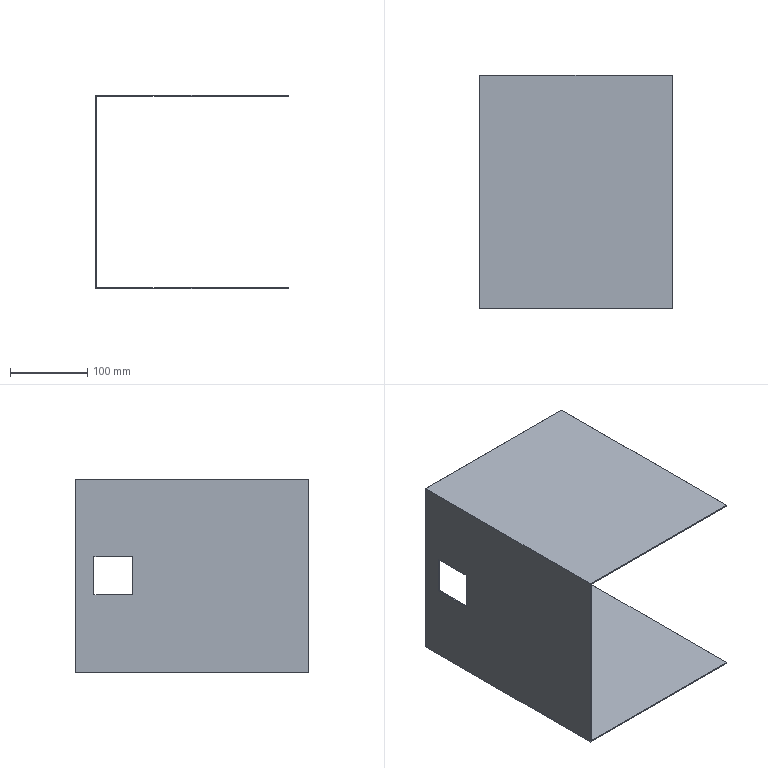Component | SolidWorks | InfraredProcessingChamber-1 | 1 solid | 14 faces | box 248.5 x 301 x 250 mm | volume 332222 mm3 | plane 14
build123d program:
from build123d import *

# Parameters (mm, degrees)
SKETCH1_W           = 250
SKETCH1_H           = 250
BOSS_EXTRUDE1_DEPTH = 301
SHELL1_T            = -1.5
SKETCH6_W           = 250
SKETCH6_H           = 301
CUT_EXTRUDE3_DEPTH  = 1.5
SKETCH7_W           = 49.25
SKETCH7_H           = 50
CUT_EXTRUDE4_DEPTH  = 1.5
SKETCH2_W           = 247
SKETCH2_H           = 247
CUT_EXTRUDE1_DEPTH  = 10


with BuildPart() as part:
    # Sketch1 → Boss-Extrude1 (new body)
    with BuildSketch(Plane(origin=(0, 0, 0), x_dir=(1, 0, 0), z_dir=(0, 1, 0))):
        Rectangle(SKETCH1_W, SKETCH1_H)
    extrude(amount=BOSS_EXTRUDE1_DEPTH)

    # Shell1
    shell1_openings = [part.faces().sort_by_distance(p)[0] for p in [
        (0, 0, 0),
    ]]
    offset(amount=SHELL1_T, openings=shell1_openings, kind=Kind.INTERSECTION)

    # Sketch6 → Cut-Extrude3 (cut)
    with BuildSketch(Plane.XY.offset(-123.5)):
        with Locations((0, 150.5)):
            Rectangle(SKETCH6_W, SKETCH6_H)
    extrude(amount=-CUT_EXTRUDE3_DEPTH, mode=Mode.SUBTRACT)

    # Sketch7 → Cut-Extrude4 (cut)
    with BuildSketch(Plane.XY.offset(125)):
        with Locations((0.375, 252)):
            Rectangle(SKETCH7_W, SKETCH7_H)
    extrude(amount=-CUT_EXTRUDE4_DEPTH, mode=Mode.SUBTRACT)

    # Sketch2 → Cut-Extrude1 (cut)
    with BuildSketch(Plane.XZ.offset(-299.5)):
        Rectangle(SKETCH2_W, SKETCH2_H)
    extrude(amount=-CUT_EXTRUDE1_DEPTH, mode=Mode.SUBTRACT)


solid = part.part

# Placed as in the assembly
solid = solid.moved(Location((175, 270, 0), (0, -90, 0)))
STEP:
#1=CARTESIAN_POINT('',(11.752,22.48,-4.862));
#2=VERTEX_POINT('',#1);
#3=CARTESIAN_POINT('',(11.752,22.48,-4.921));
#4=VERTEX_POINT('',#3);
#5=CARTESIAN_POINT('',(11.752,22.48,-4.921));
#6=DIRECTION('',(0.,0.,-1.));
#7=VECTOR('',#6,39.37);
#8=LINE('',#5,#7);
#9=EDGE_CURVE('',#2,#4,#8,.T.);
#10=ORIENTED_EDGE('',*,*,#9,.F.);
#11=CARTESIAN_POINT('',(11.752,10.63,-4.862));
#12=VERTEX_POINT('',#11);
#13=CARTESIAN_POINT('',(11.752,22.48,-4.862));
#14=DIRECTION('',(0.,-1.,0.));
#15=VECTOR('',#14,39.37);
#16=LINE('',#13,#15);
#17=EDGE_CURVE('',#2,#12,#16,.T.);
#18=ORIENTED_EDGE('',*,*,#17,.T.);
#19=CARTESIAN_POINT('',(11.752,10.63,-4.921));
#20=VERTEX_POINT('',#19);
#21=CARTESIAN_POINT('',(11.752,10.63,-4.921));
#22=DIRECTION('',(0.,0.,1.));
#23=VECTOR('',#22,39.37);
#24=LINE('',#21,#23);
#25=EDGE_CURVE('',#20,#12,#24,.T.);
#26=ORIENTED_EDGE('',*,*,#25,.F.);
#27=CARTESIAN_POINT('',(11.752,22.48,-4.921));
#28=DIRECTION('',(0.,-1.,0.));
#29=VECTOR('',#28,39.37);
#30=LINE('',#27,#29);
#31=EDGE_CURVE('',#4,#20,#30,.T.);
#32=ORIENTED_EDGE('',*,*,#31,.F.);
#33=EDGE_LOOP('',(#10,#18,#26,#32));
#34=FACE_OUTER_BOUND('',#33,.T.);
#35=CARTESIAN_POINT('',(11.752,10.63,0.));
#36=DIRECTION('',(-1.,0.,0.));
#37=DIRECTION('',(0.,0.,1.));
#38=AXIS2_PLACEMENT_3D('',#35,#36,#37);
#39=PLANE('',#38);
#40=ADVANCED_FACE('',(#34),#39,.F.);
#41=CARTESIAN_POINT('',(1.969,10.63,4.921));
#42=VERTEX_POINT('',#41);
#43=CARTESIAN_POINT('',(11.752,10.63,4.921));
#44=VERTEX_POINT('',#43);
#45=CARTESIAN_POINT('',(11.811,10.63,4.921));
#46=DIRECTION('',(1.,0.,0.));
#47=VECTOR('',#46,39.37);
#48=LINE('',#45,#47);
#49=EDGE_CURVE('',#42,#44,#48,.T.);
#50=ORIENTED_EDGE('',*,*,#49,.T.);
#51=CARTESIAN_POINT('',(11.752,22.48,4.921));
#52=VERTEX_POINT('',#51);
#53=CARTESIAN_POINT('',(11.752,22.48,4.921));
#54=DIRECTION('',(0.,1.,-0.));
#55=VECTOR('',#54,39.37);
#56=LINE('',#53,#55);
#57=EDGE_CURVE('',#44,#52,#56,.T.);
#58=ORIENTED_EDGE('',*,*,#57,.T.);
#59=CARTESIAN_POINT('',(1.969,22.48,4.921));
#60=VERTEX_POINT('',#59);
#61=CARTESIAN_POINT('',(11.811,22.48,4.921));
#62=DIRECTION('',(1.,0.,0.));
#63=VECTOR('',#62,39.37);
#64=LINE('',#61,#63);
#65=EDGE_CURVE('',#60,#52,#64,.T.);
#66=ORIENTED_EDGE('',*,*,#65,.F.);
#67=CARTESIAN_POINT('',(1.969,22.48,4.921));
#68=DIRECTION('',(0.,-1.,0.));
#69=VECTOR('',#68,39.37);
#70=LINE('',#67,#69);
#71=EDGE_CURVE('',#60,#42,#70,.T.);
#72=ORIENTED_EDGE('',*,*,#71,.T.);
#73=EDGE_LOOP('',(#50,#58,#66,#72));
#74=FACE_OUTER_BOUND('',#73,.T.);
#75=CARTESIAN_POINT('',(11.811,22.48,4.921));
#76=DIRECTION('',(0.,0.,-1.));
#77=DIRECTION('',(-1.,0.,0.));
#78=AXIS2_PLACEMENT_3D('',#75,#76,#77);
#79=PLANE('',#78);
#80=ADVANCED_FACE('',(#74),#79,.F.);
#81=CARTESIAN_POINT('',(1.969,22.48,-4.921));
#82=VERTEX_POINT('',#81);
#83=CARTESIAN_POINT('',(11.811,22.48,-4.921));
#84=DIRECTION('',(-1.,0.,0.));
#85=VECTOR('',#84,39.37);
#86=LINE('',#83,#85);
#87=EDGE_CURVE('',#4,#82,#86,.T.);
#88=ORIENTED_EDGE('',*,*,#87,.F.);
#89=ORIENTED_EDGE('',*,*,#31,.T.);
#90=CARTESIAN_POINT('',(1.969,10.63,-4.921));
#91=VERTEX_POINT('',#90);
#92=CARTESIAN_POINT('',(11.811,10.63,-4.921));
#93=DIRECTION('',(-1.,0.,0.));
#94=VECTOR('',#93,39.37);
#95=LINE('',#92,#94);
#96=EDGE_CURVE('',#20,#91,#95,.T.);
#97=ORIENTED_EDGE('',*,*,#96,.T.);
#98=CARTESIAN_POINT('',(1.969,22.48,-4.921));
#99=DIRECTION('',(0.,-1.,0.));
#100=VECTOR('',#99,39.37);
#101=LINE('',#98,#100);
#102=EDGE_CURVE('',#82,#91,#101,.T.);
#103=ORIENTED_EDGE('',*,*,#102,.F.);
#104=EDGE_LOOP('',(#88,#89,#97,#103));
#105=FACE_OUTER_BOUND('',#104,.T.);
#106=CARTESIAN_POINT('',(11.811,22.48,-4.921));
#107=DIRECTION('',(0.,0.,1.));
#108=DIRECTION('',(1.,0.,0.));
#109=AXIS2_PLACEMENT_3D('',#106,#107,#108);
#110=PLANE('',#109);
#111=ADVANCED_FACE('',(#105),#110,.F.);
#112=CARTESIAN_POINT('',(1.969,19.567,0.9843));
#113=VERTEX_POINT('',#112);
#114=CARTESIAN_POINT('',(1.969,21.535,0.9843));
#115=VERTEX_POINT('',#114);
#116=CARTESIAN_POINT('',(1.969,19.567,0.9843));
#117=DIRECTION('',(0.,1.,0.));
#118=VECTOR('',#117,39.37);
#119=LINE('',#116,#118);
#120=EDGE_CURVE('',#113,#115,#119,.T.);
#121=ORIENTED_EDGE('',*,*,#120,.F.);
#122=CARTESIAN_POINT('',(1.969,19.567,-0.9547));
#123=VERTEX_POINT('',#122);
#124=CARTESIAN_POINT('',(1.969,19.567,-0.9547));
#125=DIRECTION('',(0.,0.,1.));
#126=VECTOR('',#125,39.37);
#127=LINE('',#124,#126);
#128=EDGE_CURVE('',#123,#113,#127,.T.);
#129=ORIENTED_EDGE('',*,*,#128,.F.);
#130=CARTESIAN_POINT('',(1.969,21.535,-0.9547));
#131=VERTEX_POINT('',#130);
#132=CARTESIAN_POINT('',(1.969,21.535,-0.9547));
#133=DIRECTION('',(0.,-1.,0.));
#134=VECTOR('',#133,39.37);
#135=LINE('',#132,#134);
#136=EDGE_CURVE('',#131,#123,#135,.T.);
#137=ORIENTED_EDGE('',*,*,#136,.F.);
#138=CARTESIAN_POINT('',(1.969,21.535,0.9843));
#139=DIRECTION('',(0.,0.,-1.));
#140=VECTOR('',#139,39.37);
#141=LINE('',#138,#140);
#142=EDGE_CURVE('',#115,#131,#141,.T.);
#143=ORIENTED_EDGE('',*,*,#142,.F.);
#144=EDGE_LOOP('',(#121,#129,#137,#143));
#145=FACE_BOUND('',#144,.T.);
#146=CARTESIAN_POINT('',(1.969,10.63,-4.921));
#147=DIRECTION('',(0.,0.,1.));
#148=VECTOR('',#147,39.37);
#149=LINE('',#146,#148);
#150=EDGE_CURVE('',#91,#42,#149,.T.);
#151=ORIENTED_EDGE('',*,*,#150,.T.);
#152=ORIENTED_EDGE('',*,*,#71,.F.);
#153=CARTESIAN_POINT('',(1.969,22.48,-4.921));
#154=DIRECTION('',(0.,0.,1.));
#155=VECTOR('',#154,39.37);
#156=LINE('',#153,#155);
#157=EDGE_CURVE('',#82,#60,#156,.T.);
#158=ORIENTED_EDGE('',*,*,#157,.F.);
#159=ORIENTED_EDGE('',*,*,#102,.T.);
#160=EDGE_LOOP('',(#151,#152,#158,#159));
#161=FACE_OUTER_BOUND('',#160,.T.);
#162=CARTESIAN_POINT('',(1.969,22.48,-4.921));
#163=DIRECTION('',(1.,0.,0.));
#164=DIRECTION('',(0.,0.,-1.));
#165=AXIS2_PLACEMENT_3D('',#162,#163,#164);
#166=PLANE('',#165);
#167=ADVANCED_FACE('',(#145,#161),#166,.F.);
#168=CARTESIAN_POINT('',(2.028,22.48,-4.862));
#169=VERTEX_POINT('',#168);
#170=CARTESIAN_POINT('',(6.89,22.48,-4.862));
#171=DIRECTION('',(-1.,0.,0.));
#172=VECTOR('',#171,39.37);
#173=LINE('',#170,#172);
#174=EDGE_CURVE('',#2,#169,#173,.T.);
#175=ORIENTED_EDGE('',*,*,#174,.F.);
#176=ORIENTED_EDGE('',*,*,#9,.T.);
#177=ORIENTED_EDGE('',*,*,#87,.T.);
#178=ORIENTED_EDGE('',*,*,#157,.T.);
#179=ORIENTED_EDGE('',*,*,#65,.T.);
#180=CARTESIAN_POINT('',(11.752,22.48,4.862));
#181=VERTEX_POINT('',#180);
#182=CARTESIAN_POINT('',(11.752,22.48,-4.921));
#183=DIRECTION('',(0.,0.,-1.));
#184=VECTOR('',#183,39.37);
#185=LINE('',#182,#184);
#186=EDGE_CURVE('',#52,#181,#185,.T.);
#187=ORIENTED_EDGE('',*,*,#186,.T.);
#188=CARTESIAN_POINT('',(2.028,22.48,4.862));
#189=VERTEX_POINT('',#188);
#190=CARTESIAN_POINT('',(6.89,22.48,4.862));
#191=DIRECTION('',(1.,0.,0.));
#192=VECTOR('',#191,39.37);
#193=LINE('',#190,#192);
#194=EDGE_CURVE('',#189,#181,#193,.T.);
#195=ORIENTED_EDGE('',*,*,#194,.F.);
#196=CARTESIAN_POINT('',(2.028,22.48,0.));
#197=DIRECTION('',(0.,0.,1.));
#198=VECTOR('',#197,39.37);
#199=LINE('',#196,#198);
#200=EDGE_CURVE('',#169,#189,#199,.T.);
#201=ORIENTED_EDGE('',*,*,#200,.F.);
#202=EDGE_LOOP('',(#175,#176,#177,#178,#179,#187,#195,#201));
#203=FACE_OUTER_BOUND('',#202,.T.);
#204=CARTESIAN_POINT('',(6.89,22.48,0.));
#205=DIRECTION('',(0.,1.,0.));
#206=DIRECTION('',(-1.,0.,0.));
#207=AXIS2_PLACEMENT_3D('',#204,#205,#206);
#208=PLANE('',#207);
#209=ADVANCED_FACE('',(#203),#208,.T.);
#210=ORIENTED_EDGE('',*,*,#96,.F.);
#211=ORIENTED_EDGE('',*,*,#25,.T.);
#212=CARTESIAN_POINT('',(2.028,10.63,-4.862));
#213=VERTEX_POINT('',#212);
#214=CARTESIAN_POINT('',(11.811,10.63,-4.862));
#215=DIRECTION('',(-1.,0.,0.));
#216=VECTOR('',#215,39.37);
#217=LINE('',#214,#216);
#218=EDGE_CURVE('',#12,#213,#217,.T.);
#219=ORIENTED_EDGE('',*,*,#218,.T.);
#220=CARTESIAN_POINT('',(2.028,10.63,4.862));
#221=VERTEX_POINT('',#220);
#222=CARTESIAN_POINT('',(2.028,10.63,-4.921));
#223=DIRECTION('',(0.,0.,1.));
#224=VECTOR('',#223,39.37);
#225=LINE('',#222,#224);
#226=EDGE_CURVE('',#213,#221,#225,.T.);
#227=ORIENTED_EDGE('',*,*,#226,.T.);
#228=CARTESIAN_POINT('',(11.752,10.63,4.862));
#229=VERTEX_POINT('',#228);
#230=CARTESIAN_POINT('',(11.811,10.63,4.862));
#231=DIRECTION('',(1.,0.,0.));
#232=VECTOR('',#231,39.37);
#233=LINE('',#230,#232);
#234=EDGE_CURVE('',#221,#229,#233,.T.);
#235=ORIENTED_EDGE('',*,*,#234,.T.);
#236=CARTESIAN_POINT('',(11.752,10.63,-4.921));
#237=DIRECTION('',(0.,0.,1.));
#238=VECTOR('',#237,39.37);
#239=LINE('',#236,#238);
#240=EDGE_CURVE('',#229,#44,#239,.T.);
#241=ORIENTED_EDGE('',*,*,#240,.T.);
#242=ORIENTED_EDGE('',*,*,#49,.F.);
#243=ORIENTED_EDGE('',*,*,#150,.F.);
#244=EDGE_LOOP('',(#210,#211,#219,#227,#235,#241,#242,#243));
#245=FACE_OUTER_BOUND('',#244,.T.);
#246=CARTESIAN_POINT('',(6.89,10.63,0.));
#247=DIRECTION('',(0.,1.,0.));
#248=DIRECTION('',(-1.,0.,0.));
#249=AXIS2_PLACEMENT_3D('',#246,#247,#248);
#250=PLANE('',#249);
#251=ADVANCED_FACE('',(#245),#250,.F.);
#252=ORIENTED_EDGE('',*,*,#234,.F.);
#253=CARTESIAN_POINT('',(2.028,22.48,4.862));
#254=DIRECTION('',(0.,-1.,0.));
#255=VECTOR('',#254,39.37);
#256=LINE('',#253,#255);
#257=EDGE_CURVE('',#189,#221,#256,.T.);
#258=ORIENTED_EDGE('',*,*,#257,.F.);
#259=ORIENTED_EDGE('',*,*,#194,.T.);
#260=CARTESIAN_POINT('',(11.752,22.48,4.862));
#261=DIRECTION('',(0.,-1.,0.));
#262=VECTOR('',#261,39.37);
#263=LINE('',#260,#262);
#264=EDGE_CURVE('',#181,#229,#263,.T.);
#265=ORIENTED_EDGE('',*,*,#264,.T.);
#266=EDGE_LOOP('',(#252,#258,#259,#265));
#267=FACE_OUTER_BOUND('',#266,.T.);
#268=CARTESIAN_POINT('',(11.811,22.48,4.862));
#269=DIRECTION('',(0.,0.,-1.));
#270=DIRECTION('',(-1.,0.,0.));
#271=AXIS2_PLACEMENT_3D('',#268,#269,#270);
#272=PLANE('',#271);
#273=ADVANCED_FACE('',(#267),#272,.T.);
#274=ORIENTED_EDGE('',*,*,#218,.F.);
#275=ORIENTED_EDGE('',*,*,#17,.F.);
#276=ORIENTED_EDGE('',*,*,#174,.T.);
#277=CARTESIAN_POINT('',(2.028,22.48,-4.862));
#278=DIRECTION('',(0.,-1.,0.));
#279=VECTOR('',#278,39.37);
#280=LINE('',#277,#279);
#281=EDGE_CURVE('',#169,#213,#280,.T.);
#282=ORIENTED_EDGE('',*,*,#281,.T.);
#283=EDGE_LOOP('',(#274,#275,#276,#282));
#284=FACE_OUTER_BOUND('',#283,.T.);
#285=CARTESIAN_POINT('',(11.811,22.48,-4.862));
#286=DIRECTION('',(0.,0.,1.));
#287=DIRECTION('',(1.,0.,0.));
#288=AXIS2_PLACEMENT_3D('',#285,#286,#287);
#289=PLANE('',#288);
#290=ADVANCED_FACE('',(#284),#289,.T.);
#291=CARTESIAN_POINT('',(2.028,19.567,-0.9547));
#292=VERTEX_POINT('',#291);
#293=CARTESIAN_POINT('',(2.028,19.567,0.9843));
#294=VERTEX_POINT('',#293);
#295=CARTESIAN_POINT('',(2.028,19.567,-0.9547));
#296=DIRECTION('',(0.,0.,1.));
#297=VECTOR('',#296,39.37);
#298=LINE('',#295,#297);
#299=EDGE_CURVE('',#292,#294,#298,.T.);
#300=ORIENTED_EDGE('',*,*,#299,.T.);
#301=CARTESIAN_POINT('',(2.028,21.535,0.9843));
#302=VERTEX_POINT('',#301);
#303=CARTESIAN_POINT('',(2.028,19.567,0.9843));
#304=DIRECTION('',(0.,1.,0.));
#305=VECTOR('',#304,39.37);
#306=LINE('',#303,#305);
#307=EDGE_CURVE('',#294,#302,#306,.T.);
#308=ORIENTED_EDGE('',*,*,#307,.T.);
#309=CARTESIAN_POINT('',(2.028,21.535,-0.9547));
#310=VERTEX_POINT('',#309);
#311=CARTESIAN_POINT('',(2.028,21.535,0.9843));
#312=DIRECTION('',(0.,0.,-1.));
#313=VECTOR('',#312,39.37);
#314=LINE('',#311,#313);
#315=EDGE_CURVE('',#302,#310,#314,.T.);
#316=ORIENTED_EDGE('',*,*,#315,.T.);
#317=CARTESIAN_POINT('',(2.028,21.535,-0.9547));
#318=DIRECTION('',(0.,-1.,0.));
#319=VECTOR('',#318,39.37);
#320=LINE('',#317,#319);
#321=EDGE_CURVE('',#310,#292,#320,.T.);
#322=ORIENTED_EDGE('',*,*,#321,.T.);
#323=EDGE_LOOP('',(#300,#308,#316,#322));
#324=FACE_BOUND('',#323,.T.);
#325=ORIENTED_EDGE('',*,*,#226,.F.);
#326=ORIENTED_EDGE('',*,*,#281,.F.);
#327=ORIENTED_EDGE('',*,*,#200,.T.);
#328=ORIENTED_EDGE('',*,*,#257,.T.);
#329=EDGE_LOOP('',(#325,#326,#327,#328));
#330=FACE_OUTER_BOUND('',#329,.T.);
#331=CARTESIAN_POINT('',(2.028,22.48,-4.921));
#332=DIRECTION('',(1.,0.,0.));
#333=DIRECTION('',(0.,0.,-1.));
#334=AXIS2_PLACEMENT_3D('',#331,#332,#333);
#335=PLANE('',#334);
#336=ADVANCED_FACE('',(#324,#330),#335,.T.);
#337=ORIENTED_EDGE('',*,*,#264,.F.);
#338=ORIENTED_EDGE('',*,*,#186,.F.);
#339=ORIENTED_EDGE('',*,*,#57,.F.);
#340=ORIENTED_EDGE('',*,*,#240,.F.);
#341=EDGE_LOOP('',(#337,#338,#339,#340));
#342=FACE_OUTER_BOUND('',#341,.T.);
#343=CARTESIAN_POINT('',(11.752,10.63,0.));
#344=DIRECTION('',(-1.,0.,0.));
#345=DIRECTION('',(0.,0.,1.));
#346=AXIS2_PLACEMENT_3D('',#343,#344,#345);
#347=PLANE('',#346);
#348=ADVANCED_FACE('',(#342),#347,.F.);
#349=ORIENTED_EDGE('',*,*,#128,.T.);
#350=CARTESIAN_POINT('',(2.028,19.567,0.9843));
#351=DIRECTION('',(-1.,0.,0.));
#352=VECTOR('',#351,39.37);
#353=LINE('',#350,#352);
#354=EDGE_CURVE('',#294,#113,#353,.T.);
#355=ORIENTED_EDGE('',*,*,#354,.F.);
#356=ORIENTED_EDGE('',*,*,#299,.F.);
#357=CARTESIAN_POINT('',(2.028,19.567,-0.9547));
#358=DIRECTION('',(-1.,0.,0.));
#359=VECTOR('',#358,39.37);
#360=LINE('',#357,#359);
#361=EDGE_CURVE('',#292,#123,#360,.T.);
#362=ORIENTED_EDGE('',*,*,#361,.T.);
#363=EDGE_LOOP('',(#349,#355,#356,#362));
#364=FACE_OUTER_BOUND('',#363,.T.);
#365=CARTESIAN_POINT('',(2.028,19.567,-0.9547));
#366=DIRECTION('',(0.,-1.,0.));
#367=DIRECTION('',(1.,0.,0.));
#368=AXIS2_PLACEMENT_3D('',#365,#366,#367);
#369=PLANE('',#368);
#370=ADVANCED_FACE('',(#364),#369,.F.);
#371=ORIENTED_EDGE('',*,*,#136,.T.);
#372=ORIENTED_EDGE('',*,*,#361,.F.);
#373=ORIENTED_EDGE('',*,*,#321,.F.);
#374=CARTESIAN_POINT('',(2.028,21.535,-0.9547));
#375=DIRECTION('',(-1.,0.,0.));
#376=VECTOR('',#375,39.37);
#377=LINE('',#374,#376);
#378=EDGE_CURVE('',#310,#131,#377,.T.);
#379=ORIENTED_EDGE('',*,*,#378,.T.);
#380=EDGE_LOOP('',(#371,#372,#373,#379));
#381=FACE_OUTER_BOUND('',#380,.T.);
#382=CARTESIAN_POINT('',(2.028,21.535,-0.9547));
#383=DIRECTION('',(0.,-0.,-1.));
#384=DIRECTION('',(0.,-1.,0.));
#385=AXIS2_PLACEMENT_3D('',#382,#383,#384);
#386=PLANE('',#385);
#387=ADVANCED_FACE('',(#381),#386,.F.);
#388=ORIENTED_EDGE('',*,*,#142,.T.);
#389=ORIENTED_EDGE('',*,*,#378,.F.);
#390=ORIENTED_EDGE('',*,*,#315,.F.);
#391=CARTESIAN_POINT('',(2.028,21.535,0.9843));
#392=DIRECTION('',(-1.,0.,0.));
#393=VECTOR('',#392,39.37);
#394=LINE('',#391,#393);
#395=EDGE_CURVE('',#302,#115,#394,.T.);
#396=ORIENTED_EDGE('',*,*,#395,.T.);
#397=EDGE_LOOP('',(#388,#389,#390,#396));
#398=FACE_OUTER_BOUND('',#397,.T.);
#399=CARTESIAN_POINT('',(2.028,21.535,0.9843));
#400=DIRECTION('',(0.,1.,0.));
#401=DIRECTION('',(-1.,0.,0.));
#402=AXIS2_PLACEMENT_3D('',#399,#400,#401);
#403=PLANE('',#402);
#404=ADVANCED_FACE('',(#398),#403,.F.);
#405=ORIENTED_EDGE('',*,*,#120,.T.);
#406=ORIENTED_EDGE('',*,*,#395,.F.);
#407=ORIENTED_EDGE('',*,*,#307,.F.);
#408=ORIENTED_EDGE('',*,*,#354,.T.);
#409=EDGE_LOOP('',(#405,#406,#407,#408));
#410=FACE_OUTER_BOUND('',#409,.T.);
#411=CARTESIAN_POINT('',(2.028,19.567,0.9843));
#412=DIRECTION('',(0.,0.,1.));
#413=DIRECTION('',(1.,0.,0.));
#414=AXIS2_PLACEMENT_3D('',#411,#412,#413);
#415=PLANE('',#414);
#416=ADVANCED_FACE('',(#410),#415,.F.);
#417=CLOSED_SHELL('',(#40,#80,#111,#167,#209,#251,#273,#290,#336,#348,#370,#387,#404,#416));
#418=MANIFOLD_SOLID_BREP('',#417);
#419=CARTESIAN_POINT('',(0.,0.,0.));
#420=DIRECTION('',(0.,0.,1.));
#421=DIRECTION('',(1.,0.,0.));
#422=AXIS2_PLACEMENT_3D('',#419,#420,#421);
#423=(LENGTH_UNIT()NAMED_UNIT(*)SI_UNIT($,.METRE.));
#424=LENGTH_MEASURE_WITH_UNIT(LENGTH_MEASURE(0.0254),#423);
#425=DIMENSIONAL_EXPONENTS(1.,0.,0.,0.,0.,0.,0.);
#426=(CONVERSION_BASED_UNIT('',#424)LENGTH_UNIT()NAMED_UNIT(#425));
#427=UNCERTAINTY_MEASURE_WITH_UNIT(LENGTH_MEASURE(0.00001),#426,'','');
#428=(NAMED_UNIT(*)PLANE_ANGLE_UNIT()SI_UNIT($,.RADIAN.));
#429=(NAMED_UNIT(*)SI_UNIT($,.STERADIAN.)SOLID_ANGLE_UNIT());
#430=(GEOMETRIC_REPRESENTATION_CONTEXT(3)GLOBAL_UNCERTAINTY_ASSIGNED_CONTEXT((#427))GLOBAL_UNIT_ASSIGNED_CONTEXT((#426,#428,#429))REPRESENTATION_CONTEXT('',''));
#431=ADVANCED_BREP_SHAPE_REPRESENTATION('',(#418,#422),#430);
#432=COLOUR_RGB('',0.7922,0.8196,0.9333);
#433=FILL_AREA_STYLE_COLOUR('',#432);
#434=FILL_AREA_STYLE('',(#433));
#435=SURFACE_STYLE_FILL_AREA(#434);
#436=SURFACE_SIDE_STYLE('',(#435));
#437=SURFACE_STYLE_USAGE(.BOTH.,#436);
#438=PRESENTATION_STYLE_ASSIGNMENT((#437));
#439=STYLED_ITEM('',(#438),#418);
#440=PRESENTATION_LAYER_ASSIGNMENT('','',(#439));
#441=(LENGTH_UNIT()NAMED_UNIT(*)SI_UNIT($,.METRE.));
#442=LENGTH_MEASURE_WITH_UNIT(LENGTH_MEASURE(0.0254),#441);
#443=DIMENSIONAL_EXPONENTS(1.,0.,0.,0.,0.,0.,0.);
#444=(CONVERSION_BASED_UNIT('',#442)LENGTH_UNIT()NAMED_UNIT(#443));
#445=UNCERTAINTY_MEASURE_WITH_UNIT(LENGTH_MEASURE(0.00001),#444,'','');
#446=(NAMED_UNIT(*)PLANE_ANGLE_UNIT()SI_UNIT($,.RADIAN.));
#447=(NAMED_UNIT(*)SI_UNIT($,.STERADIAN.)SOLID_ANGLE_UNIT());
#448=(GEOMETRIC_REPRESENTATION_CONTEXT(3)GLOBAL_UNCERTAINTY_ASSIGNED_CONTEXT((#445))GLOBAL_UNIT_ASSIGNED_CONTEXT((#444,#446,#447))REPRESENTATION_CONTEXT('',''));
#449=MECHANICAL_DESIGN_GEOMETRIC_PRESENTATION_REPRESENTATION('',(#439),#448);